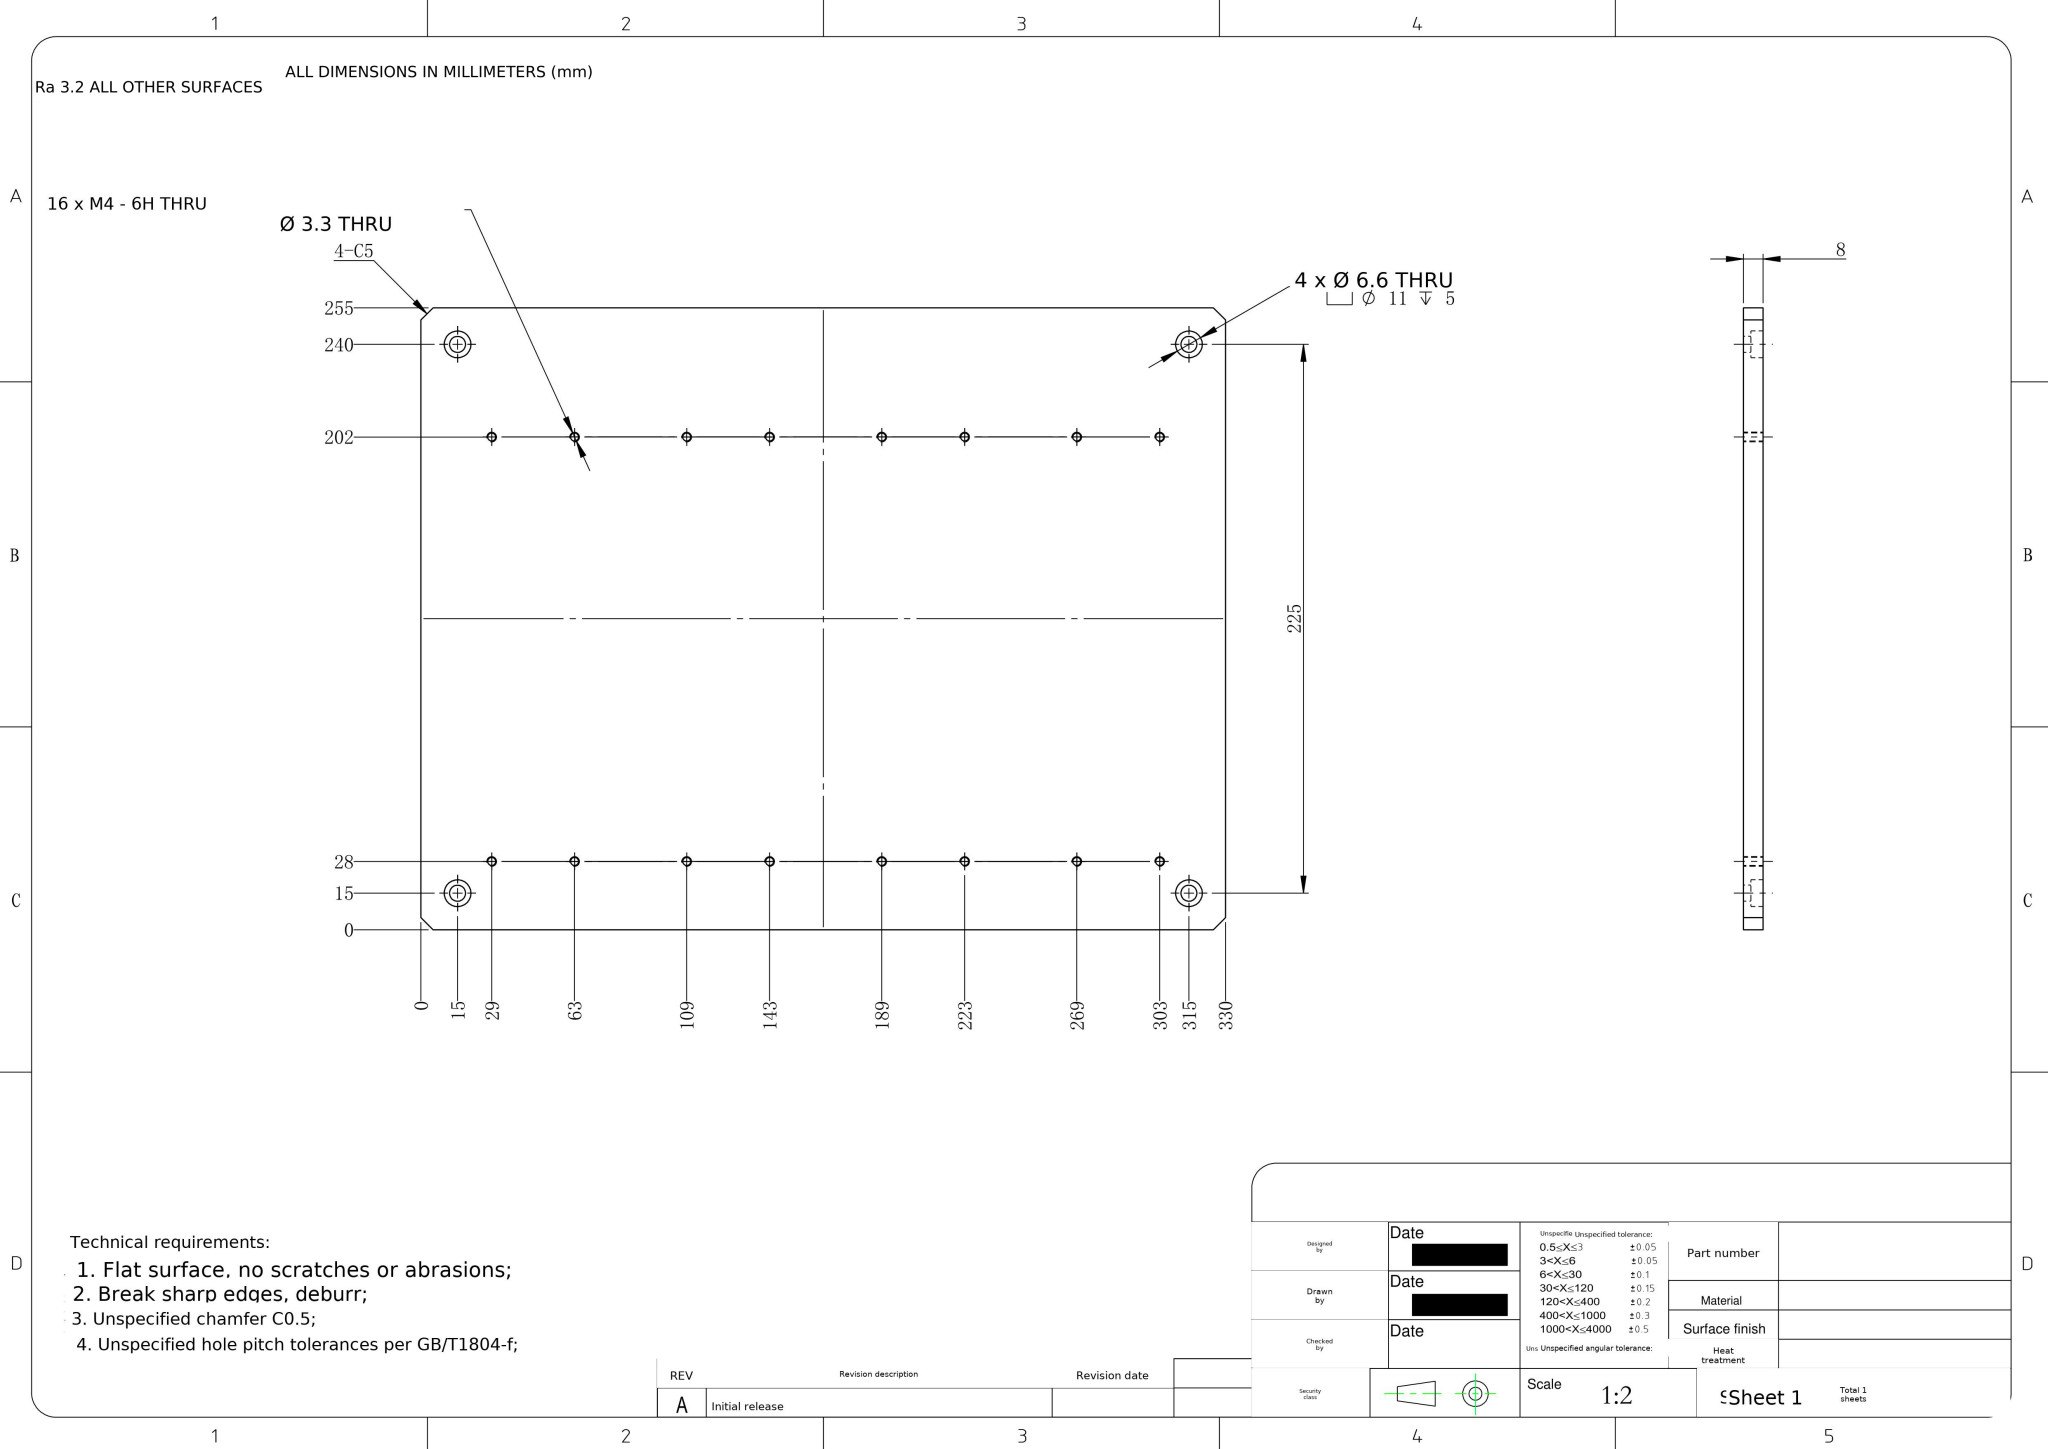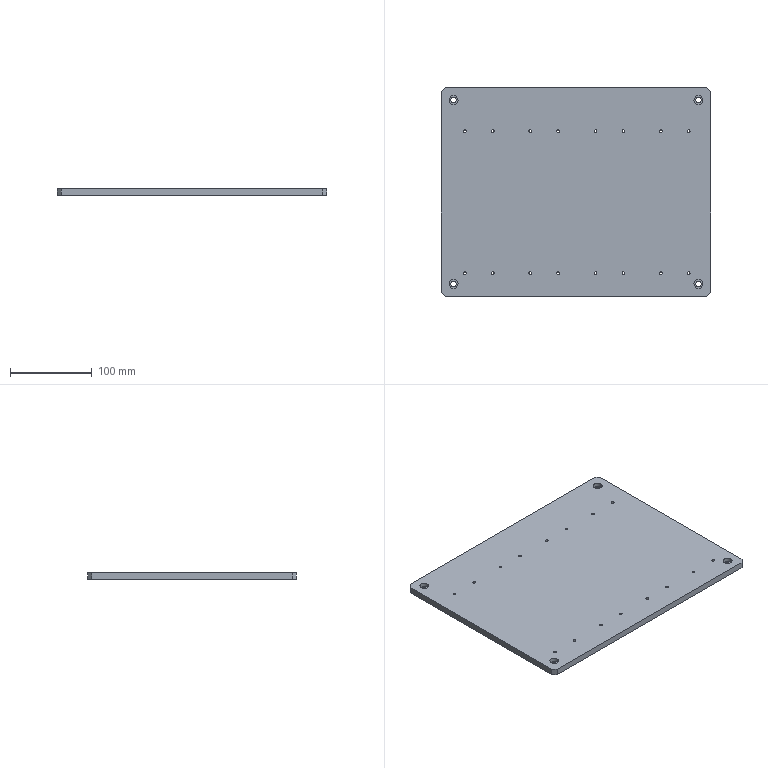Part | NX | mm | 1 solid | 62 faces | box 330 x 255 x 8 mm | volume 669394 mm3 | cylinder 48 | plane 14 | commonest cylinder face diameters 3.3 x32 11 x8 6.6 x8